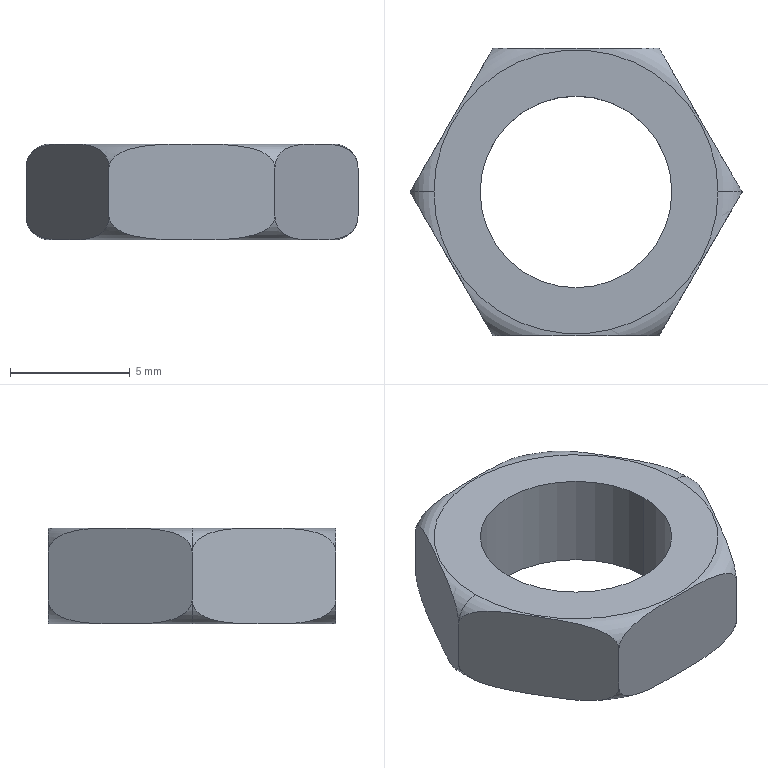Component | SolidWorks | F-YBXFJFA-RB0806-1_F-YBXFJFA-RB0806_Rb-Nut-2 | 1 solid | 14 faces | box 13.86 x 12 x 4 mm | volume 296 mm3 | plane 8 | torus 4 | cylinder 2 | commonest cylinder face diameters 8 x2
STEP:
#1=COLOUR_RGB('',0.7922,0.8196,0.9333);
#2=FILL_AREA_STYLE_COLOUR('',#1);
#3=FILL_AREA_STYLE('',(#2));
#4=SURFACE_STYLE_FILL_AREA(#3);
#5=SURFACE_SIDE_STYLE('',(#4));
#6=SURFACE_STYLE_USAGE(.BOTH.,#5);
#7=PRESENTATION_STYLE_ASSIGNMENT((#6));
#8=CARTESIAN_POINT('',(10.954,12.172,1.83));
#9=VERTEX_POINT('',#8);
#10=CARTESIAN_POINT('',(10.487,12.172,1.83));
#11=VERTEX_POINT('',#10);
#12=CARTESIAN_POINT('',(10.721,12.172,1.83));
#13=DIRECTION('',(0.,0.,1.));
#14=DIRECTION('',(1.,0.,0.));
#15=AXIS2_PLACEMENT_3D('',#12,#13,#14);
#16=CIRCLE('',#15,0.2334);
#17=EDGE_CURVE('',#9,#11,#16,.T.);
#18=ORIENTED_EDGE('',*,*,#17,.T.);
#19=CARTESIAN_POINT('',(10.448,12.172,1.869));
#20=VERTEX_POINT('',#19);
#21=CARTESIAN_POINT('',(10.487,12.172,1.869));
#22=DIRECTION('',(0.,1.,0.));
#23=DIRECTION('',(-1.,0.,0.));
#24=AXIS2_PLACEMENT_3D('',#21,#22,#23);
#25=CIRCLE('',#24,0.03937);
#26=EDGE_CURVE('',#11,#20,#25,.T.);
#27=ORIENTED_EDGE('',*,*,#26,.T.);
#28=CARTESIAN_POINT('',(10.584,12.408,1.869));
#29=VERTEX_POINT('',#28);
#30=CARTESIAN_POINT('',(10.448,12.172,1.869));
#31=CARTESIAN_POINT('',(10.448,12.172,1.866));
#32=CARTESIAN_POINT('',(10.448,12.173,1.863));
#33=CARTESIAN_POINT('',(10.45,12.175,1.857));
#34=CARTESIAN_POINT('',(10.451,12.177,1.854));
#35=CARTESIAN_POINT('',(10.453,12.181,1.85));
#36=CARTESIAN_POINT('',(10.454,12.183,1.848));
#37=CARTESIAN_POINT('',(10.457,12.188,1.845));
#38=CARTESIAN_POINT('',(10.458,12.19,1.843));
#39=CARTESIAN_POINT('',(10.463,12.198,1.839));
#40=CARTESIAN_POINT('',(10.466,12.203,1.837));
#41=CARTESIAN_POINT('',(10.472,12.214,1.835));
#42=CARTESIAN_POINT('',(10.475,12.219,1.833));
#43=CARTESIAN_POINT('',(10.484,12.236,1.831));
#44=CARTESIAN_POINT('',(10.491,12.247,1.831));
#45=CARTESIAN_POINT('',(10.503,12.269,1.83));
#46=CARTESIAN_POINT('',(10.51,12.28,1.83));
#47=CARTESIAN_POINT('',(10.523,12.301,1.83));
#48=CARTESIAN_POINT('',(10.529,12.312,1.83));
#49=CARTESIAN_POINT('',(10.542,12.334,1.831));
#50=CARTESIAN_POINT('',(10.548,12.345,1.831));
#51=CARTESIAN_POINT('',(10.557,12.362,1.834));
#52=CARTESIAN_POINT('',(10.56,12.367,1.835));
#53=CARTESIAN_POINT('',(10.567,12.378,1.837));
#54=CARTESIAN_POINT('',(10.57,12.383,1.839));
#55=CARTESIAN_POINT('',(10.575,12.393,1.845));
#56=CARTESIAN_POINT('',(10.578,12.398,1.848));
#57=CARTESIAN_POINT('',(10.582,12.404,1.855));
#58=CARTESIAN_POINT('',(10.582,12.405,1.857));
#59=CARTESIAN_POINT('',(10.584,12.408,1.863));
#60=CARTESIAN_POINT('',(10.584,12.408,1.866));
#61=CARTESIAN_POINT('',(10.584,12.408,1.869));
#62=B_SPLINE_CURVE_WITH_KNOTS('',3,(#30,#31,#32,#33,#34,#35,#36,#37,#38,#39,#40,#41,#42,#43,#44,#45,#46,#47,#48,#49,#50,#51,#52,#53,#54,#55,#56,#57,#58,#59,#60,#61),.UNSPECIFIED.,.F.,.F.,(4,2,2,2,2,2,2,2,2,2,2,2,2,2,2,4),(0.0000002,0.0002437,0.0004871,0.0007306,0.0009741,0.001461,0.001948,0.002922,0.003896,0.00487,0.005843,0.00633,0.006817,0.007304,0.007548,0.007791),.UNSPECIFIED.);
#63=EDGE_CURVE('',#20,#29,#62,.T.);
#64=ORIENTED_EDGE('',*,*,#63,.T.);
#65=CARTESIAN_POINT('',(10.857,12.408,1.869));
#66=VERTEX_POINT('',#65);
#67=CARTESIAN_POINT('',(10.584,12.408,1.869));
#68=CARTESIAN_POINT('',(10.584,12.408,1.866));
#69=CARTESIAN_POINT('',(10.585,12.408,1.863));
#70=CARTESIAN_POINT('',(10.588,12.408,1.857));
#71=CARTESIAN_POINT('',(10.59,12.408,1.855));
#72=CARTESIAN_POINT('',(10.594,12.408,1.85));
#73=CARTESIAN_POINT('',(10.597,12.408,1.848));
#74=CARTESIAN_POINT('',(10.602,12.408,1.845));
#75=CARTESIAN_POINT('',(10.605,12.408,1.843));
#76=CARTESIAN_POINT('',(10.614,12.408,1.839));
#77=CARTESIAN_POINT('',(10.62,12.408,1.837));
#78=CARTESIAN_POINT('',(10.632,12.408,1.835));
#79=CARTESIAN_POINT('',(10.638,12.408,1.834));
#80=CARTESIAN_POINT('',(10.657,12.408,1.831));
#81=CARTESIAN_POINT('',(10.67,12.408,1.831));
#82=CARTESIAN_POINT('',(10.695,12.408,1.83));
#83=CARTESIAN_POINT('',(10.708,12.408,1.83));
#84=CARTESIAN_POINT('',(10.733,12.408,1.83));
#85=CARTESIAN_POINT('',(10.746,12.408,1.83));
#86=CARTESIAN_POINT('',(10.771,12.408,1.831));
#87=CARTESIAN_POINT('',(10.784,12.408,1.831));
#88=CARTESIAN_POINT('',(10.803,12.408,1.833));
#89=CARTESIAN_POINT('',(10.809,12.408,1.835));
#90=CARTESIAN_POINT('',(10.821,12.408,1.837));
#91=CARTESIAN_POINT('',(10.827,12.408,1.839));
#92=CARTESIAN_POINT('',(10.839,12.408,1.844));
#93=CARTESIAN_POINT('',(10.845,12.408,1.848));
#94=CARTESIAN_POINT('',(10.851,12.408,1.854));
#95=CARTESIAN_POINT('',(10.853,12.408,1.857));
#96=CARTESIAN_POINT('',(10.856,12.408,1.863));
#97=CARTESIAN_POINT('',(10.857,12.408,1.866));
#98=CARTESIAN_POINT('',(10.857,12.408,1.869));
#99=B_SPLINE_CURVE_WITH_KNOTS('',3,(#67,#68,#69,#70,#71,#72,#73,#74,#75,#76,#77,#78,#79,#80,#81,#82,#83,#84,#85,#86,#87,#88,#89,#90,#91,#92,#93,#94,#95,#96,#97,#98),.UNSPECIFIED.,.F.,.F.,(4,2,2,2,2,2,2,2,2,2,2,2,2,2,2,4),(0.01157,0.01181,0.01205,0.01229,0.01253,0.01302,0.0135,0.01446,0.01543,0.0164,0.01736,0.01784,0.01833,0.01881,0.01905,0.01929),.UNSPECIFIED.);
#100=EDGE_CURVE('',#29,#66,#99,.T.);
#101=ORIENTED_EDGE('',*,*,#100,.T.);
#102=CARTESIAN_POINT('',(10.993,12.172,1.869));
#103=VERTEX_POINT('',#102);
#104=CARTESIAN_POINT('',(10.857,12.408,1.869));
#105=CARTESIAN_POINT('',(10.857,12.408,1.866));
#106=CARTESIAN_POINT('',(10.857,12.408,1.863));
#107=CARTESIAN_POINT('',(10.859,12.405,1.857));
#108=CARTESIAN_POINT('',(10.86,12.404,1.854));
#109=CARTESIAN_POINT('',(10.862,12.4,1.85));
#110=CARTESIAN_POINT('',(10.863,12.397,1.848));
#111=CARTESIAN_POINT('',(10.866,12.393,1.845));
#112=CARTESIAN_POINT('',(10.868,12.39,1.843));
#113=CARTESIAN_POINT('',(10.872,12.383,1.839));
#114=CARTESIAN_POINT('',(10.875,12.377,1.837));
#115=CARTESIAN_POINT('',(10.881,12.367,1.835));
#116=CARTESIAN_POINT('',(10.884,12.361,1.833));
#117=CARTESIAN_POINT('',(10.894,12.345,1.831));
#118=CARTESIAN_POINT('',(10.9,12.334,1.831));
#119=CARTESIAN_POINT('',(10.913,12.312,1.83));
#120=CARTESIAN_POINT('',(10.919,12.301,1.83));
#121=CARTESIAN_POINT('',(10.932,12.279,1.83));
#122=CARTESIAN_POINT('',(10.938,12.268,1.83));
#123=CARTESIAN_POINT('',(10.951,12.246,1.831));
#124=CARTESIAN_POINT('',(10.957,12.235,1.831));
#125=CARTESIAN_POINT('',(10.966,12.219,1.834));
#126=CARTESIAN_POINT('',(10.97,12.214,1.835));
#127=CARTESIAN_POINT('',(10.976,12.203,1.837));
#128=CARTESIAN_POINT('',(10.979,12.198,1.839));
#129=CARTESIAN_POINT('',(10.985,12.188,1.845));
#130=CARTESIAN_POINT('',(10.987,12.183,1.848));
#131=CARTESIAN_POINT('',(10.991,12.177,1.855));
#132=CARTESIAN_POINT('',(10.992,12.175,1.857));
#133=CARTESIAN_POINT('',(10.993,12.173,1.863));
#134=CARTESIAN_POINT('',(10.993,12.172,1.866));
#135=CARTESIAN_POINT('',(10.993,12.172,1.869));
#136=B_SPLINE_CURVE_WITH_KNOTS('',3,(#104,#105,#106,#107,#108,#109,#110,#111,#112,#113,#114,#115,#116,#117,#118,#119,#120,#121,#122,#123,#124,#125,#126,#127,#128,#129,#130,#131,#132,#133,#134,#135),.UNSPECIFIED.,.F.,.F.,(4,2,2,2,2,2,2,2,2,2,2,2,2,2,2,4),(0.0000002,0.0002437,0.0004871,0.0007306,0.0009741,0.001461,0.001948,0.002922,0.003896,0.00487,0.005843,0.00633,0.006817,0.007304,0.007548,0.007791),.UNSPECIFIED.);
#137=EDGE_CURVE('',#66,#103,#136,.T.);
#138=ORIENTED_EDGE('',*,*,#137,.T.);
#139=CARTESIAN_POINT('',(10.954,12.172,1.869));
#140=DIRECTION('',(0.,-1.,0.));
#141=DIRECTION('',(0.,0.,-1.));
#142=AXIS2_PLACEMENT_3D('',#139,#140,#141);
#143=CIRCLE('',#142,0.03937);
#144=EDGE_CURVE('',#9,#103,#143,.T.);
#145=ORIENTED_EDGE('',*,*,#144,.F.);
#146=EDGE_LOOP('',(#18,#27,#64,#101,#138,#145));
#147=FACE_OUTER_BOUND('',#146,.T.);
#148=CARTESIAN_POINT('',(10.721,12.172,1.869));
#149=DIRECTION('',(0.,0.,1.));
#150=DIRECTION('',(1.,0.,0.));
#151=AXIS2_PLACEMENT_3D('',#148,#149,#150);
#152=TOROIDAL_SURFACE('',#151,0.2334,0.03937);
#153=ADVANCED_FACE('',(#147),#152,.T.);
#154=CARTESIAN_POINT('',(10.584,12.408,1.948));
#155=VERTEX_POINT('',#154);
#156=CARTESIAN_POINT('',(10.448,12.172,1.948));
#157=VERTEX_POINT('',#156);
#158=CARTESIAN_POINT('',(10.584,12.408,1.948));
#159=CARTESIAN_POINT('',(10.584,12.408,1.951));
#160=CARTESIAN_POINT('',(10.584,12.408,1.954));
#161=CARTESIAN_POINT('',(10.582,12.405,1.96));
#162=CARTESIAN_POINT('',(10.581,12.404,1.963));
#163=CARTESIAN_POINT('',(10.579,12.4,1.967));
#164=CARTESIAN_POINT('',(10.578,12.397,1.969));
#165=CARTESIAN_POINT('',(10.575,12.393,1.973));
#166=CARTESIAN_POINT('',(10.574,12.39,1.974));
#167=CARTESIAN_POINT('',(10.569,12.383,1.978));
#168=CARTESIAN_POINT('',(10.566,12.377,1.98));
#169=CARTESIAN_POINT('',(10.56,12.367,1.983));
#170=CARTESIAN_POINT('',(10.557,12.361,1.984));
#171=CARTESIAN_POINT('',(10.548,12.345,1.986));
#172=CARTESIAN_POINT('',(10.541,12.334,1.987));
#173=CARTESIAN_POINT('',(10.529,12.312,1.987));
#174=CARTESIAN_POINT('',(10.522,12.301,1.987));
#175=CARTESIAN_POINT('',(10.51,12.279,1.987));
#176=CARTESIAN_POINT('',(10.503,12.268,1.987));
#177=CARTESIAN_POINT('',(10.491,12.246,1.987));
#178=CARTESIAN_POINT('',(10.484,12.235,1.986));
#179=CARTESIAN_POINT('',(10.475,12.219,1.984));
#180=CARTESIAN_POINT('',(10.472,12.214,1.983));
#181=CARTESIAN_POINT('',(10.466,12.203,1.98));
#182=CARTESIAN_POINT('',(10.463,12.198,1.978));
#183=CARTESIAN_POINT('',(10.457,12.188,1.973));
#184=CARTESIAN_POINT('',(10.454,12.183,1.969));
#185=CARTESIAN_POINT('',(10.451,12.177,1.963));
#186=CARTESIAN_POINT('',(10.45,12.175,1.96));
#187=CARTESIAN_POINT('',(10.448,12.173,1.954));
#188=CARTESIAN_POINT('',(10.448,12.172,1.951));
#189=CARTESIAN_POINT('',(10.448,12.172,1.948));
#190=B_SPLINE_CURVE_WITH_KNOTS('',3,(#158,#159,#160,#161,#162,#163,#164,#165,#166,#167,#168,#169,#170,#171,#172,#173,#174,#175,#176,#177,#178,#179,#180,#181,#182,#183,#184,#185,#186,#187,#188,#189),.UNSPECIFIED.,.F.,.F.,(4,2,2,2,2,2,2,2,2,2,2,2,2,2,2,4),(0.0000002,0.0002437,0.0004871,0.0007306,0.0009741,0.001461,0.001948,0.002922,0.003896,0.00487,0.005843,0.00633,0.006817,0.007304,0.007548,0.007791),.UNSPECIFIED.);
#191=EDGE_CURVE('',#155,#157,#190,.T.);
#192=ORIENTED_EDGE('',*,*,#191,.T.);
#193=CARTESIAN_POINT('',(10.487,12.172,1.987));
#194=VERTEX_POINT('',#193);
#195=CARTESIAN_POINT('',(10.487,12.172,1.948));
#196=DIRECTION('',(0.,1.,0.));
#197=DIRECTION('',(-1.,0.,0.));
#198=AXIS2_PLACEMENT_3D('',#195,#196,#197);
#199=CIRCLE('',#198,0.03937);
#200=EDGE_CURVE('',#157,#194,#199,.T.);
#201=ORIENTED_EDGE('',*,*,#200,.T.);
#202=CARTESIAN_POINT('',(10.954,12.172,1.987));
#203=VERTEX_POINT('',#202);
#204=CARTESIAN_POINT('',(10.721,12.172,1.987));
#205=DIRECTION('',(0.,0.,1.));
#206=DIRECTION('',(1.,0.,0.));
#207=AXIS2_PLACEMENT_3D('',#204,#205,#206);
#208=CIRCLE('',#207,0.2334);
#209=EDGE_CURVE('',#203,#194,#208,.T.);
#210=ORIENTED_EDGE('',*,*,#209,.F.);
#211=CARTESIAN_POINT('',(10.993,12.172,1.948));
#212=VERTEX_POINT('',#211);
#213=CARTESIAN_POINT('',(10.954,12.172,1.948));
#214=DIRECTION('',(0.,-1.,0.));
#215=DIRECTION('',(0.,0.,-1.));
#216=AXIS2_PLACEMENT_3D('',#213,#214,#215);
#217=CIRCLE('',#216,0.03937);
#218=EDGE_CURVE('',#212,#203,#217,.T.);
#219=ORIENTED_EDGE('',*,*,#218,.F.);
#220=CARTESIAN_POINT('',(10.857,12.408,1.948));
#221=VERTEX_POINT('',#220);
#222=CARTESIAN_POINT('',(10.993,12.172,1.948));
#223=CARTESIAN_POINT('',(10.993,12.172,1.951));
#224=CARTESIAN_POINT('',(10.993,12.173,1.954));
#225=CARTESIAN_POINT('',(10.992,12.175,1.96));
#226=CARTESIAN_POINT('',(10.991,12.177,1.963));
#227=CARTESIAN_POINT('',(10.988,12.181,1.967));
#228=CARTESIAN_POINT('',(10.987,12.183,1.969));
#229=CARTESIAN_POINT('',(10.984,12.188,1.973));
#230=CARTESIAN_POINT('',(10.983,12.19,1.974));
#231=CARTESIAN_POINT('',(10.979,12.198,1.978));
#232=CARTESIAN_POINT('',(10.976,12.203,1.98));
#233=CARTESIAN_POINT('',(10.969,12.214,1.983));
#234=CARTESIAN_POINT('',(10.966,12.219,1.984));
#235=CARTESIAN_POINT('',(10.957,12.236,1.986));
#236=CARTESIAN_POINT('',(10.951,12.247,1.987));
#237=CARTESIAN_POINT('',(10.938,12.269,1.987));
#238=CARTESIAN_POINT('',(10.932,12.28,1.987));
#239=CARTESIAN_POINT('',(10.919,12.301,1.987));
#240=CARTESIAN_POINT('',(10.913,12.312,1.987));
#241=CARTESIAN_POINT('',(10.9,12.334,1.987));
#242=CARTESIAN_POINT('',(10.894,12.345,1.986));
#243=CARTESIAN_POINT('',(10.884,12.362,1.984));
#244=CARTESIAN_POINT('',(10.881,12.367,1.983));
#245=CARTESIAN_POINT('',(10.875,12.378,1.98));
#246=CARTESIAN_POINT('',(10.872,12.383,1.978));
#247=CARTESIAN_POINT('',(10.866,12.393,1.973));
#248=CARTESIAN_POINT('',(10.863,12.398,1.969));
#249=CARTESIAN_POINT('',(10.86,12.404,1.963));
#250=CARTESIAN_POINT('',(10.859,12.405,1.96));
#251=CARTESIAN_POINT('',(10.857,12.408,1.954));
#252=CARTESIAN_POINT('',(10.857,12.408,1.951));
#253=CARTESIAN_POINT('',(10.857,12.408,1.948));
#254=B_SPLINE_CURVE_WITH_KNOTS('',3,(#222,#223,#224,#225,#226,#227,#228,#229,#230,#231,#232,#233,#234,#235,#236,#237,#238,#239,#240,#241,#242,#243,#244,#245,#246,#247,#248,#249,#250,#251,#252,#253),.UNSPECIFIED.,.F.,.F.,(4,2,2,2,2,2,2,2,2,2,2,2,2,2,2,4),(0.0000002,0.0002437,0.0004871,0.0007306,0.0009741,0.001461,0.001948,0.002922,0.003896,0.00487,0.005843,0.00633,0.006817,0.007304,0.007548,0.007791),.UNSPECIFIED.);
#255=EDGE_CURVE('',#212,#221,#254,.T.);
#256=ORIENTED_EDGE('',*,*,#255,.T.);
#257=CARTESIAN_POINT('',(10.857,12.408,1.948));
#258=CARTESIAN_POINT('',(10.857,12.408,1.951));
#259=CARTESIAN_POINT('',(10.856,12.408,1.954));
#260=CARTESIAN_POINT('',(10.853,12.408,1.96));
#261=CARTESIAN_POINT('',(10.851,12.408,1.963));
#262=CARTESIAN_POINT('',(10.847,12.408,1.967));
#263=CARTESIAN_POINT('',(10.844,12.408,1.969));
#264=CARTESIAN_POINT('',(10.839,12.408,1.973));
#265=CARTESIAN_POINT('',(10.836,12.408,1.974));
#266=CARTESIAN_POINT('',(10.828,12.408,1.978));
#267=CARTESIAN_POINT('',(10.821,12.408,1.98));
#268=CARTESIAN_POINT('',(10.809,12.408,1.983));
#269=CARTESIAN_POINT('',(10.803,12.408,1.984));
#270=CARTESIAN_POINT('',(10.784,12.408,1.986));
#271=CARTESIAN_POINT('',(10.772,12.408,1.987));
#272=CARTESIAN_POINT('',(10.746,12.408,1.987));
#273=CARTESIAN_POINT('',(10.734,12.408,1.987));
#274=CARTESIAN_POINT('',(10.708,12.408,1.987));
#275=CARTESIAN_POINT('',(10.696,12.408,1.987));
#276=CARTESIAN_POINT('',(10.67,12.408,1.987));
#277=CARTESIAN_POINT('',(10.658,12.408,1.986));
#278=CARTESIAN_POINT('',(10.639,12.408,1.984));
#279=CARTESIAN_POINT('',(10.632,12.408,1.983));
#280=CARTESIAN_POINT('',(10.62,12.408,1.98));
#281=CARTESIAN_POINT('',(10.614,12.408,1.978));
#282=CARTESIAN_POINT('',(10.602,12.408,1.973));
#283=CARTESIAN_POINT('',(10.597,12.408,1.97));
#284=CARTESIAN_POINT('',(10.59,12.408,1.963));
#285=CARTESIAN_POINT('',(10.588,12.408,1.96));
#286=CARTESIAN_POINT('',(10.585,12.408,1.954));
#287=CARTESIAN_POINT('',(10.584,12.408,1.951));
#288=CARTESIAN_POINT('',(10.584,12.408,1.948));
#289=B_SPLINE_CURVE_WITH_KNOTS('',3,(#257,#258,#259,#260,#261,#262,#263,#264,#265,#266,#267,#268,#269,#270,#271,#272,#273,#274,#275,#276,#277,#278,#279,#280,#281,#282,#283,#284,#285,#286,#287,#288),.UNSPECIFIED.,.F.,.F.,(4,2,2,2,2,2,2,2,2,2,2,2,2,2,2,4),(0.01157,0.01181,0.01205,0.01229,0.01253,0.01302,0.0135,0.01446,0.01543,0.0164,0.01736,0.01784,0.01833,0.01881,0.01905,0.01929),.UNSPECIFIED.);
#290=EDGE_CURVE('',#221,#155,#289,.T.);
#291=ORIENTED_EDGE('',*,*,#290,.T.);
#292=EDGE_LOOP('',(#192,#201,#210,#219,#256,#291));
#293=FACE_OUTER_BOUND('',#292,.T.);
#294=CARTESIAN_POINT('',(10.721,12.172,1.948));
#295=DIRECTION('',(0.,0.,1.));
#296=DIRECTION('',(1.,0.,0.));
#297=AXIS2_PLACEMENT_3D('',#294,#295,#296);
#298=TOROIDAL_SURFACE('',#297,0.2334,0.03937);
#299=ADVANCED_FACE('',(#293),#298,.T.);
#300=CARTESIAN_POINT('',(10.563,12.172,1.987));
#301=VERTEX_POINT('',#300);
#302=CARTESIAN_POINT('',(10.878,12.172,1.987));
#303=VERTEX_POINT('',#302);
#304=CARTESIAN_POINT('',(10.721,12.172,1.987));
#305=DIRECTION('',(0.,0.,1.));
#306=DIRECTION('',(1.,0.,0.));
#307=AXIS2_PLACEMENT_3D('',#304,#305,#306);
#308=CIRCLE('',#307,0.1575);
#309=EDGE_CURVE('',#301,#303,#308,.T.);
#310=ORIENTED_EDGE('',*,*,#309,.T.);
#311=CARTESIAN_POINT('',(10.878,12.172,1.83));
#312=VERTEX_POINT('',#311);
#313=CARTESIAN_POINT('',(10.878,12.172,1.987));
#314=DIRECTION('',(0.,0.,-1.));
#315=VECTOR('',#314,39.37);
#316=LINE('',#313,#315);
#317=EDGE_CURVE('',#303,#312,#316,.T.);
#318=ORIENTED_EDGE('',*,*,#317,.T.);
#319=CARTESIAN_POINT('',(10.563,12.172,1.83));
#320=VERTEX_POINT('',#319);
#321=CARTESIAN_POINT('',(10.721,12.172,1.83));
#322=DIRECTION('',(0.,0.,1.));
#323=DIRECTION('',(1.,0.,0.));
#324=AXIS2_PLACEMENT_3D('',#321,#322,#323);
#325=CIRCLE('',#324,0.1575);
#326=EDGE_CURVE('',#320,#312,#325,.T.);
#327=ORIENTED_EDGE('',*,*,#326,.F.);
#328=CARTESIAN_POINT('',(10.563,12.172,1.987));
#329=DIRECTION('',(0.,0.,-1.));
#330=VECTOR('',#329,39.37);
#331=LINE('',#328,#330);
#332=EDGE_CURVE('',#301,#320,#331,.T.);
#333=ORIENTED_EDGE('',*,*,#332,.F.);
#334=EDGE_LOOP('',(#310,#318,#327,#333));
#335=FACE_OUTER_BOUND('',#334,.T.);
#336=CARTESIAN_POINT('',(10.721,12.172,1.987));
#337=DIRECTION('',(0.,0.,-1.));
#338=DIRECTION('',(-1.,0.,0.));
#339=AXIS2_PLACEMENT_3D('',#336,#337,#338);
#340=CYLINDRICAL_SURFACE('',#339,0.1575);
#341=ADVANCED_FACE('',(#335),#340,.F.);
#342=CARTESIAN_POINT('',(10.857,11.936,1.869));
#343=VERTEX_POINT('',#342);
#344=CARTESIAN_POINT('',(10.993,12.172,1.869));
#345=CARTESIAN_POINT('',(10.993,12.172,1.866));
#346=CARTESIAN_POINT('',(10.993,12.172,1.863));
#347=CARTESIAN_POINT('',(10.992,12.169,1.857));
#348=CARTESIAN_POINT('',(10.991,12.167,1.854));
#349=CARTESIAN_POINT('',(10.988,12.163,1.85));
#350=CARTESIAN_POINT('',(10.987,12.161,1.848));
#351=CARTESIAN_POINT('',(10.984,12.157,1.845));
#352=CARTESIAN_POINT('',(10.983,12.154,1.843));
#353=CARTESIAN_POINT('',(10.979,12.147,1.839));
#354=CARTESIAN_POINT('',(10.976,12.141,1.837));
#355=CARTESIAN_POINT('',(10.969,12.131,1.835));
#356=CARTESIAN_POINT('',(10.966,12.125,1.833));
#357=CARTESIAN_POINT('',(10.957,12.109,1.831));
#358=CARTESIAN_POINT('',(10.951,12.098,1.831));
#359=CARTESIAN_POINT('',(10.938,12.076,1.83));
#360=CARTESIAN_POINT('',(10.932,12.065,1.83));
#361=CARTESIAN_POINT('',(10.919,12.043,1.83));
#362=CARTESIAN_POINT('',(10.913,12.032,1.83));
#363=CARTESIAN_POINT('',(10.9,12.01,1.831));
#364=CARTESIAN_POINT('',(10.894,11.999,1.831));
#365=CARTESIAN_POINT('',(10.884,11.983,1.834));
#366=CARTESIAN_POINT('',(10.881,11.977,1.835));
#367=CARTESIAN_POINT('',(10.875,11.967,1.837));
#368=CARTESIAN_POINT('',(10.872,11.962,1.839));
#369=CARTESIAN_POINT('',(10.866,11.951,1.845));
#370=CARTESIAN_POINT('',(10.863,11.947,1.848));
#371=CARTESIAN_POINT('',(10.86,11.941,1.855));
#372=CARTESIAN_POINT('',(10.859,11.939,1.857));
#373=CARTESIAN_POINT('',(10.857,11.937,1.863));
#374=CARTESIAN_POINT('',(10.857,11.936,1.866));
#375=CARTESIAN_POINT('',(10.857,11.936,1.869));
#376=B_SPLINE_CURVE_WITH_KNOTS('',3,(#344,#345,#346,#347,#348,#349,#350,#351,#352,#353,#354,#355,#356,#357,#358,#359,#360,#361,#362,#363,#364,#365,#366,#367,#368,#369,#370,#371,#372,#373,#374,#375),.UNSPECIFIED.,.F.,.F.,(4,2,2,2,2,2,2,2,2,2,2,2,2,2,2,4),(0.0000002,0.0002437,0.0004871,0.0007306,0.0009741,0.001461,0.001948,0.002922,0.003896,0.00487,0.005843,0.00633,0.006817,0.007304,0.007548,0.007791),.UNSPECIFIED.);
#377=EDGE_CURVE('',#103,#343,#376,.T.);
#378=ORIENTED_EDGE('',*,*,#377,.F.);
#379=CARTESIAN_POINT('',(10.993,12.172,1.987));
#380=DIRECTION('',(0.,0.,-1.));
#381=VECTOR('',#380,39.37);
#382=LINE('',#379,#381);
#383=EDGE_CURVE('',#212,#103,#382,.T.);
#384=ORIENTED_EDGE('',*,*,#383,.F.);
#385=CARTESIAN_POINT('',(10.857,11.936,1.948));
#386=VERTEX_POINT('',#385);
#387=CARTESIAN_POINT('',(10.857,11.936,1.948));
#388=CARTESIAN_POINT('',(10.857,11.936,1.951));
#389=CARTESIAN_POINT('',(10.857,11.937,1.954));
#390=CARTESIAN_POINT('',(10.859,11.939,1.96));
#391=CARTESIAN_POINT('',(10.86,11.941,1.963));
#392=CARTESIAN_POINT('',(10.862,11.945,1.967));
#393=CARTESIAN_POINT('',(10.863,11.947,1.969));
#394=CARTESIAN_POINT('',(10.866,11.952,1.973));
#395=CARTESIAN_POINT('',(10.868,11.954,1.974));
#396=CARTESIAN_POINT('',(10.872,11.962,1.978));
#397=CARTESIAN_POINT('',(10.875,11.967,1.98));
#398=CARTESIAN_POINT('',(10.881,11.978,1.983));
#399=CARTESIAN_POINT('',(10.884,11.983,1.984));
#400=CARTESIAN_POINT('',(10.894,11.999,1.986));
#401=CARTESIAN_POINT('',(10.9,12.01,1.987));
#402=CARTESIAN_POINT('',(10.913,12.032,1.987));
#403=CARTESIAN_POINT('',(10.919,12.043,1.987));
#404=CARTESIAN_POINT('',(10.932,12.065,1.987));
#405=CARTESIAN_POINT('',(10.938,12.076,1.987));
#406=CARTESIAN_POINT('',(10.951,12.098,1.987));
#407=CARTESIAN_POINT('',(10.957,12.109,1.986));
#408=CARTESIAN_POINT('',(10.966,12.125,1.984));
#409=CARTESIAN_POINT('',(10.97,12.131,1.983));
#410=CARTESIAN_POINT('',(10.976,12.142,1.98));
#411=CARTESIAN_POINT('',(10.979,12.147,1.978));
#412=CARTESIAN_POINT('',(10.985,12.157,1.973));
#413=CARTESIAN_POINT('',(10.987,12.162,1.969));
#414=CARTESIAN_POINT('',(10.991,12.167,1.963));
#415=CARTESIAN_POINT('',(10.992,12.169,1.96));
#416=CARTESIAN_POINT('',(10.993,12.172,1.954));
#417=CARTESIAN_POINT('',(10.993,12.172,1.951));
#418=CARTESIAN_POINT('',(10.993,12.172,1.948));
#419=B_SPLINE_CURVE_WITH_KNOTS('',3,(#387,#388,#389,#390,#391,#392,#393,#394,#395,#396,#397,#398,#399,#400,#401,#402,#403,#404,#405,#406,#407,#408,#409,#410,#411,#412,#413,#414,#415,#416,#417,#418),.UNSPECIFIED.,.F.,.F.,(4,2,2,2,2,2,2,2,2,2,2,2,2,2,2,4),(0.0000002,0.0002437,0.0004871,0.0007306,0.0009741,0.001461,0.001948,0.002922,0.003896,0.00487,0.005843,0.00633,0.006817,0.007304,0.007548,0.007791),.UNSPECIFIED.);
#420=EDGE_CURVE('',#386,#212,#419,.T.);
#421=ORIENTED_EDGE('',*,*,#420,.F.);
#422=CARTESIAN_POINT('',(10.857,11.936,1.987));
#423=DIRECTION('',(0.,0.,-1.));
#424=VECTOR('',#423,39.37);
#425=LINE('',#422,#424);
#426=EDGE_CURVE('',#386,#343,#425,.T.);
#427=ORIENTED_EDGE('',*,*,#426,.T.);
#428=EDGE_LOOP('',(#378,#384,#421,#427));
#429=FACE_OUTER_BOUND('',#428,.T.);
#430=CARTESIAN_POINT('',(10.857,11.936,1.987));
#431=DIRECTION('',(-0.866,0.5,0.));
#432=DIRECTION('',(-0.5,-0.866,0.));
#433=AXIS2_PLACEMENT_3D('',#430,#431,#432);
#434=PLANE('',#433);
#435=ADVANCED_FACE('',(#429),#434,.F.);
#436=ORIENTED_EDGE('',*,*,#137,.F.);
#437=CARTESIAN_POINT('',(10.857,12.408,1.987));
#438=DIRECTION('',(0.,0.,-1.));
#439=VECTOR('',#438,39.37);
#440=LINE('',#437,#439);
#441=EDGE_CURVE('',#221,#66,#440,.T.);
#442=ORIENTED_EDGE('',*,*,#441,.F.);
#443=ORIENTED_EDGE('',*,*,#255,.F.);
#444=ORIENTED_EDGE('',*,*,#383,.T.);
#445=EDGE_LOOP('',(#436,#442,#443,#444));
#446=FACE_OUTER_BOUND('',#445,.T.);
#447=CARTESIAN_POINT('',(10.993,12.172,1.987));
#448=DIRECTION('',(-0.866,-0.5,0.));
#449=DIRECTION('',(0.5,-0.866,0.));
#450=AXIS2_PLACEMENT_3D('',#447,#448,#449);
#451=PLANE('',#450);
#452=ADVANCED_FACE('',(#446),#451,.F.);
#453=ORIENTED_EDGE('',*,*,#100,.F.);
#454=CARTESIAN_POINT('',(10.584,12.408,1.987));
#455=DIRECTION('',(0.,0.,-1.));
#456=VECTOR('',#455,39.37);
#457=LINE('',#454,#456);
#458=EDGE_CURVE('',#155,#29,#457,.T.);
#459=ORIENTED_EDGE('',*,*,#458,.F.);
#460=ORIENTED_EDGE('',*,*,#290,.F.);
#461=ORIENTED_EDGE('',*,*,#441,.T.);
#462=EDGE_LOOP('',(#453,#459,#460,#461));
#463=FACE_OUTER_BOUND('',#462,.T.);
#464=CARTESIAN_POINT('',(10.857,12.408,1.987));
#465=DIRECTION('',(0.,-1.,0.));
#466=DIRECTION('',(0.,0.,-1.));
#467=AXIS2_PLACEMENT_3D('',#464,#465,#466);
#468=PLANE('',#467);
#469=ADVANCED_FACE('',(#463),#468,.F.);
#470=ORIENTED_EDGE('',*,*,#63,.F.);
#471=CARTESIAN_POINT('',(10.448,12.172,1.987));
#472=DIRECTION('',(0.,0.,-1.));
#473=VECTOR('',#472,39.37);
#474=LINE('',#471,#473);
#475=EDGE_CURVE('',#157,#20,#474,.T.);
#476=ORIENTED_EDGE('',*,*,#475,.F.);
#477=ORIENTED_EDGE('',*,*,#191,.F.);
#478=ORIENTED_EDGE('',*,*,#458,.T.);
#479=EDGE_LOOP('',(#470,#476,#477,#478));
#480=FACE_OUTER_BOUND('',#479,.T.);
#481=CARTESIAN_POINT('',(10.584,12.408,1.987));
#482=DIRECTION('',(0.866,-0.5,0.));
#483=DIRECTION('',(0.5,0.866,0.));
#484=AXIS2_PLACEMENT_3D('',#481,#482,#483);
#485=PLANE('',#484);
#486=ADVANCED_FACE('',(#480),#485,.F.);
#487=CARTESIAN_POINT('',(10.584,11.936,1.869));
#488=VERTEX_POINT('',#487);
#489=CARTESIAN_POINT('',(10.584,11.936,1.869));
#490=CARTESIAN_POINT('',(10.584,11.936,1.866));
#491=CARTESIAN_POINT('',(10.584,11.937,1.863));
#492=CARTESIAN_POINT('',(10.582,11.939,1.857));
#493=CARTESIAN_POINT('',(10.581,11.941,1.854));
#494=CARTESIAN_POINT('',(10.579,11.945,1.85));
#495=CARTESIAN_POINT('',(10.578,11.947,1.848));
#496=CARTESIAN_POINT('',(10.575,11.952,1.845));
#497=CARTESIAN_POINT('',(10.574,11.954,1.843));
#498=CARTESIAN_POINT('',(10.569,11.962,1.839));
#499=CARTESIAN_POINT('',(10.566,11.967,1.837));
#500=CARTESIAN_POINT('',(10.56,11.978,1.835));
#501=CARTESIAN_POINT('',(10.557,11.983,1.833));
#502=CARTESIAN_POINT('',(10.548,11.999,1.831));
#503=CARTESIAN_POINT('',(10.541,12.01,1.831));
#504=CARTESIAN_POINT('',(10.529,12.032,1.83));
#505=CARTESIAN_POINT('',(10.522,12.043,1.83));
#506=CARTESIAN_POINT('',(10.51,12.065,1.83));
#507=CARTESIAN_POINT('',(10.503,12.076,1.83));
#508=CARTESIAN_POINT('',(10.491,12.098,1.831));
#509=CARTESIAN_POINT('',(10.484,12.109,1.831));
#510=CARTESIAN_POINT('',(10.475,12.125,1.834));
#511=CARTESIAN_POINT('',(10.472,12.131,1.835));
#512=CARTESIAN_POINT('',(10.466,12.142,1.837));
#513=CARTESIAN_POINT('',(10.463,12.147,1.839));
#514=CARTESIAN_POINT('',(10.457,12.157,1.845));
#515=CARTESIAN_POINT('',(10.454,12.162,1.848));
#516=CARTESIAN_POINT('',(10.451,12.167,1.855));
#517=CARTESIAN_POINT('',(10.45,12.169,1.857));
#518=CARTESIAN_POINT('',(10.448,12.172,1.863));
#519=CARTESIAN_POINT('',(10.448,12.172,1.866));
#520=CARTESIAN_POINT('',(10.448,12.172,1.869));
#521=B_SPLINE_CURVE_WITH_KNOTS('',3,(#489,#490,#491,#492,#493,#494,#495,#496,#497,#498,#499,#500,#501,#502,#503,#504,#505,#506,#507,#508,#509,#510,#511,#512,#513,#514,#515,#516,#517,#518,#519,#520),.UNSPECIFIED.,.F.,.F.,(4,2,2,2,2,2,2,2,2,2,2,2,2,2,2,4),(0.0000002,0.0002437,0.0004871,0.0007306,0.0009741,0.001461,0.001948,0.002922,0.003896,0.00487,0.005843,0.00633,0.006817,0.007304,0.007548,0.007791),.UNSPECIFIED.);
#522=EDGE_CURVE('',#488,#20,#521,.T.);
#523=ORIENTED_EDGE('',*,*,#522,.F.);
#524=CARTESIAN_POINT('',(10.584,11.936,1.948));
#525=VERTEX_POINT('',#524);
#526=CARTESIAN_POINT('',(10.584,11.936,1.987));
#527=DIRECTION('',(0.,0.,-1.));
#528=VECTOR('',#527,39.37);
#529=LINE('',#526,#528);
#530=EDGE_CURVE('',#525,#488,#529,.T.);
#531=ORIENTED_EDGE('',*,*,#530,.F.);
#532=CARTESIAN_POINT('',(10.448,12.172,1.948));
#533=CARTESIAN_POINT('',(10.448,12.172,1.951));
#534=CARTESIAN_POINT('',(10.448,12.172,1.954));
#535=CARTESIAN_POINT('',(10.45,12.169,1.96));
#536=CARTESIAN_POINT('',(10.451,12.167,1.963));
#537=CARTESIAN_POINT('',(10.453,12.163,1.967));
#538=CARTESIAN_POINT('',(10.454,12.161,1.969));
#539=CARTESIAN_POINT('',(10.457,12.157,1.973));
#540=CARTESIAN_POINT('',(10.458,12.154,1.974));
#541=CARTESIAN_POINT('',(10.463,12.147,1.978));
#542=CARTESIAN_POINT('',(10.466,12.141,1.98));
#543=CARTESIAN_POINT('',(10.472,12.131,1.983));
#544=CARTESIAN_POINT('',(10.475,12.125,1.984));
#545=CARTESIAN_POINT('',(10.484,12.109,1.986));
#546=CARTESIAN_POINT('',(10.491,12.098,1.987));
#547=CARTESIAN_POINT('',(10.503,12.076,1.987));
#548=CARTESIAN_POINT('',(10.51,12.065,1.987));
#549=CARTESIAN_POINT('',(10.523,12.043,1.987));
#550=CARTESIAN_POINT('',(10.529,12.032,1.987));
#551=CARTESIAN_POINT('',(10.542,12.01,1.987));
#552=CARTESIAN_POINT('',(10.548,11.999,1.986));
#553=CARTESIAN_POINT('',(10.557,11.983,1.984));
#554=CARTESIAN_POINT('',(10.56,11.977,1.983));
#555=CARTESIAN_POINT('',(10.567,11.967,1.98));
#556=CARTESIAN_POINT('',(10.57,11.962,1.978));
#557=CARTESIAN_POINT('',(10.575,11.951,1.973));
#558=CARTESIAN_POINT('',(10.578,11.947,1.969));
#559=CARTESIAN_POINT('',(10.582,11.941,1.963));
#560=CARTESIAN_POINT('',(10.582,11.939,1.96));
#561=CARTESIAN_POINT('',(10.584,11.937,1.954));
#562=CARTESIAN_POINT('',(10.584,11.936,1.951));
#563=CARTESIAN_POINT('',(10.584,11.936,1.948));
#564=B_SPLINE_CURVE_WITH_KNOTS('',3,(#532,#533,#534,#535,#536,#537,#538,#539,#540,#541,#542,#543,#544,#545,#546,#547,#548,#549,#550,#551,#552,#553,#554,#555,#556,#557,#558,#559,#560,#561,#562,#563),.UNSPECIFIED.,.F.,.F.,(4,2,2,2,2,2,2,2,2,2,2,2,2,2,2,4),(0.0000002,0.0002437,0.0004871,0.0007306,0.0009741,0.001461,0.001948,0.002922,0.003896,0.00487,0.005843,0.00633,0.006817,0.007304,0.007548,0.007791),.UNSPECIFIED.);
#565=EDGE_CURVE('',#157,#525,#564,.T.);
#566=ORIENTED_EDGE('',*,*,#565,.F.);
#567=ORIENTED_EDGE('',*,*,#475,.T.);
#568=EDGE_LOOP('',(#523,#531,#566,#567));
#569=FACE_OUTER_BOUND('',#568,.T.);
#570=CARTESIAN_POINT('',(10.448,12.172,1.987));
#571=DIRECTION('',(0.866,0.5,0.));
#572=DIRECTION('',(-0.5,0.866,0.));
#573=AXIS2_PLACEMENT_3D('',#570,#571,#572);
#574=PLANE('',#573);
#575=ADVANCED_FACE('',(#569),#574,.F.);
#576=CARTESIAN_POINT('',(10.857,11.936,1.869));
#577=CARTESIAN_POINT('',(10.857,11.936,1.866));
#578=CARTESIAN_POINT('',(10.856,11.936,1.863));
#579=CARTESIAN_POINT('',(10.853,11.936,1.857));
#580=CARTESIAN_POINT('',(10.851,11.936,1.855));
#581=CARTESIAN_POINT('',(10.847,11.936,1.85));
#582=CARTESIAN_POINT('',(10.844,11.936,1.848));
#583=CARTESIAN_POINT('',(10.839,11.936,1.845));
#584=CARTESIAN_POINT('',(10.836,11.936,1.843));
#585=CARTESIAN_POINT('',(10.828,11.936,1.839));
#586=CARTESIAN_POINT('',(10.821,11.936,1.837));
#587=CARTESIAN_POINT('',(10.809,11.936,1.835));
#588=CARTESIAN_POINT('',(10.803,11.936,1.834));
#589=CARTESIAN_POINT('',(10.784,11.936,1.831));
#590=CARTESIAN_POINT('',(10.772,11.936,1.831));
#591=CARTESIAN_POINT('',(10.746,11.936,1.83));
#592=CARTESIAN_POINT('',(10.734,11.936,1.83));
#593=CARTESIAN_POINT('',(10.708,11.936,1.83));
#594=CARTESIAN_POINT('',(10.696,11.936,1.83));
#595=CARTESIAN_POINT('',(10.67,11.936,1.831));
#596=CARTESIAN_POINT('',(10.658,11.936,1.831));
#597=CARTESIAN_POINT('',(10.639,11.936,1.833));
#598=CARTESIAN_POINT('',(10.632,11.936,1.835));
#599=CARTESIAN_POINT('',(10.62,11.936,1.837));
#600=CARTESIAN_POINT('',(10.614,11.936,1.839));
#601=CARTESIAN_POINT('',(10.602,11.936,1.844));
#602=CARTESIAN_POINT('',(10.597,11.936,1.848));
#603=CARTESIAN_POINT('',(10.59,11.936,1.854));
#604=CARTESIAN_POINT('',(10.588,11.936,1.857));
#605=CARTESIAN_POINT('',(10.585,11.936,1.863));
#606=CARTESIAN_POINT('',(10.584,11.936,1.866));
#607=CARTESIAN_POINT('',(10.584,11.936,1.869));
#608=B_SPLINE_CURVE_WITH_KNOTS('',3,(#576,#577,#578,#579,#580,#581,#582,#583,#584,#585,#586,#587,#588,#589,#590,#591,#592,#593,#594,#595,#596,#597,#598,#599,#600,#601,#602,#603,#604,#605,#606,#607),.UNSPECIFIED.,.F.,.F.,(4,2,2,2,2,2,2,2,2,2,2,2,2,2,2,4),(0.01157,0.01181,0.01205,0.01229,0.01253,0.01302,0.0135,0.01446,0.01543,0.0164,0.01736,0.01784,0.01833,0.01881,0.01905,0.01929),.UNSPECIFIED.);
#609=EDGE_CURVE('',#343,#488,#608,.T.);
#610=ORIENTED_EDGE('',*,*,#609,.F.);
#611=ORIENTED_EDGE('',*,*,#426,.F.);
#612=CARTESIAN_POINT('',(10.584,11.936,1.948));
#613=CARTESIAN_POINT('',(10.584,11.936,1.951));
#614=CARTESIAN_POINT('',(10.585,11.936,1.954));
#615=CARTESIAN_POINT('',(10.588,11.936,1.96));
#616=CARTESIAN_POINT('',(10.59,11.936,1.963));
#617=CARTESIAN_POINT('',(10.594,11.936,1.967));
#618=CARTESIAN_POINT('',(10.597,11.936,1.969));
#619=CARTESIAN_POINT('',(10.602,11.936,1.973));
#620=CARTESIAN_POINT('',(10.605,11.936,1.974));
#621=CARTESIAN_POINT('',(10.614,11.936,1.978));
#622=CARTESIAN_POINT('',(10.62,11.936,1.98));
#623=CARTESIAN_POINT('',(10.632,11.936,1.983));
#624=CARTESIAN_POINT('',(10.638,11.936,1.984));
#625=CARTESIAN_POINT('',(10.657,11.936,1.986));
#626=CARTESIAN_POINT('',(10.67,11.936,1.987));
#627=CARTESIAN_POINT('',(10.695,11.936,1.987));
#628=CARTESIAN_POINT('',(10.708,11.936,1.987));
#629=CARTESIAN_POINT('',(10.733,11.936,1.987));
#630=CARTESIAN_POINT('',(10.746,11.936,1.987));
#631=CARTESIAN_POINT('',(10.771,11.936,1.987));
#632=CARTESIAN_POINT('',(10.784,11.936,1.986));
#633=CARTESIAN_POINT('',(10.803,11.936,1.984));
#634=CARTESIAN_POINT('',(10.809,11.936,1.983));
#635=CARTESIAN_POINT('',(10.821,11.936,1.98));
#636=CARTESIAN_POINT('',(10.827,11.936,1.978));
#637=CARTESIAN_POINT('',(10.839,11.936,1.973));
#638=CARTESIAN_POINT('',(10.845,11.936,1.97));
#639=CARTESIAN_POINT('',(10.851,11.936,1.963));
#640=CARTESIAN_POINT('',(10.853,11.936,1.96));
#641=CARTESIAN_POINT('',(10.856,11.936,1.954));
#642=CARTESIAN_POINT('',(10.857,11.936,1.951));
#643=CARTESIAN_POINT('',(10.857,11.936,1.948));
#644=B_SPLINE_CURVE_WITH_KNOTS('',3,(#612,#613,#614,#615,#616,#617,#618,#619,#620,#621,#622,#623,#624,#625,#626,#627,#628,#629,#630,#631,#632,#633,#634,#635,#636,#637,#638,#639,#640,#641,#642,#643),.UNSPECIFIED.,.F.,.F.,(4,2,2,2,2,2,2,2,2,2,2,2,2,2,2,4),(0.01157,0.01181,0.01205,0.01229,0.01253,0.01302,0.0135,0.01446,0.01543,0.0164,0.01736,0.01784,0.01833,0.01881,0.01905,0.01929),.UNSPECIFIED.);
#645=EDGE_CURVE('',#525,#386,#644,.T.);
#646=ORIENTED_EDGE('',*,*,#645,.F.);
#647=ORIENTED_EDGE('',*,*,#530,.T.);
#648=EDGE_LOOP('',(#610,#611,#646,#647));
#649=FACE_OUTER_BOUND('',#648,.T.);
#650=CARTESIAN_POINT('',(10.584,11.936,1.987));
#651=DIRECTION('',(-0.,1.,0.));
#652=DIRECTION('',(-1.,-0.,0.));
#653=AXIS2_PLACEMENT_3D('',#650,#651,#652);
#654=PLANE('',#653);
#655=ADVANCED_FACE('',(#649),#654,.F.);
#656=ORIENTED_EDGE('',*,*,#326,.T.);
#657=CARTESIAN_POINT('',(10.721,12.172,1.83));
#658=DIRECTION('',(0.,0.,1.));
#659=DIRECTION('',(1.,0.,0.));
#660=AXIS2_PLACEMENT_3D('',#657,#658,#659);
#661=CIRCLE('',#660,0.1575);
#662=EDGE_CURVE('',#312,#320,#661,.T.);
#663=ORIENTED_EDGE('',*,*,#662,.T.);
#664=EDGE_LOOP('',(#656,#663));
#665=FACE_BOUND('',#664,.T.);
#666=ORIENTED_EDGE('',*,*,#17,.F.);
#667=CARTESIAN_POINT('',(10.721,12.172,1.83));
#668=DIRECTION('',(0.,0.,1.));
#669=DIRECTION('',(1.,0.,0.));
#670=AXIS2_PLACEMENT_3D('',#667,#668,#669);
#671=CIRCLE('',#670,0.2334);
#672=EDGE_CURVE('',#11,#9,#671,.T.);
#673=ORIENTED_EDGE('',*,*,#672,.F.);
#674=EDGE_LOOP('',(#666,#673));
#675=FACE_OUTER_BOUND('',#674,.T.);
#676=CARTESIAN_POINT('',(11.13,12.408,1.83));
#677=DIRECTION('',(0.,0.,1.));
#678=DIRECTION('',(1.,0.,0.));
#679=AXIS2_PLACEMENT_3D('',#676,#677,#678);
#680=PLANE('',#679);
#681=ADVANCED_FACE('',(#665,#675),#680,.F.);
#682=ORIENTED_EDGE('',*,*,#309,.F.);
#683=CARTESIAN_POINT('',(10.721,12.172,1.987));
#684=DIRECTION('',(0.,0.,1.));
#685=DIRECTION('',(1.,0.,0.));
#686=AXIS2_PLACEMENT_3D('',#683,#684,#685);
#687=CIRCLE('',#686,0.1575);
#688=EDGE_CURVE('',#303,#301,#687,.T.);
#689=ORIENTED_EDGE('',*,*,#688,.F.);
#690=EDGE_LOOP('',(#682,#689));
#691=FACE_BOUND('',#690,.T.);
#692=ORIENTED_EDGE('',*,*,#209,.T.);
#693=CARTESIAN_POINT('',(10.721,12.172,1.987));
#694=DIRECTION('',(0.,0.,1.));
#695=DIRECTION('',(1.,0.,0.));
#696=AXIS2_PLACEMENT_3D('',#693,#694,#695);
#697=CIRCLE('',#696,0.2334);
#698=EDGE_CURVE('',#194,#203,#697,.T.);
#699=ORIENTED_EDGE('',*,*,#698,.T.);
#700=EDGE_LOOP('',(#692,#699));
#701=FACE_OUTER_BOUND('',#700,.T.);
#702=CARTESIAN_POINT('',(11.13,12.408,1.987));
#703=DIRECTION('',(0.,0.,1.));
#704=DIRECTION('',(1.,0.,0.));
#705=AXIS2_PLACEMENT_3D('',#702,#703,#704);
#706=PLANE('',#705);
#707=ADVANCED_FACE('',(#691,#701),#706,.T.);
#708=ORIENTED_EDGE('',*,*,#317,.F.);
#709=ORIENTED_EDGE('',*,*,#688,.T.);
#710=ORIENTED_EDGE('',*,*,#332,.T.);
#711=ORIENTED_EDGE('',*,*,#662,.F.);
#712=EDGE_LOOP('',(#708,#709,#710,#711));
#713=FACE_OUTER_BOUND('',#712,.T.);
#714=CARTESIAN_POINT('',(10.721,12.172,1.987));
#715=DIRECTION('',(0.,0.,-1.));
#716=DIRECTION('',(-1.,0.,0.));
#717=AXIS2_PLACEMENT_3D('',#714,#715,#716);
#718=CYLINDRICAL_SURFACE('',#717,0.1575);
#719=ADVANCED_FACE('',(#713),#718,.F.);
#720=ORIENTED_EDGE('',*,*,#200,.F.);
#721=ORIENTED_EDGE('',*,*,#565,.T.);
#722=ORIENTED_EDGE('',*,*,#645,.T.);
#723=ORIENTED_EDGE('',*,*,#420,.T.);
#724=ORIENTED_EDGE('',*,*,#218,.T.);
#725=ORIENTED_EDGE('',*,*,#698,.F.);
#726=EDGE_LOOP('',(#720,#721,#722,#723,#724,#725));
#727=FACE_OUTER_BOUND('',#726,.T.);
#728=CARTESIAN_POINT('',(10.721,12.172,1.948));
#729=DIRECTION('',(0.,0.,1.));
#730=DIRECTION('',(1.,0.,0.));
#731=AXIS2_PLACEMENT_3D('',#728,#729,#730);
#732=TOROIDAL_SURFACE('',#731,0.2334,0.03937);
#733=ADVANCED_FACE('',(#727),#732,.T.);
#734=ORIENTED_EDGE('',*,*,#26,.F.);
#735=ORIENTED_EDGE('',*,*,#672,.T.);
#736=ORIENTED_EDGE('',*,*,#144,.T.);
#737=ORIENTED_EDGE('',*,*,#377,.T.);
#738=ORIENTED_EDGE('',*,*,#609,.T.);
#739=ORIENTED_EDGE('',*,*,#522,.T.);
#740=EDGE_LOOP('',(#734,#735,#736,#737,#738,#739));
#741=FACE_OUTER_BOUND('',#740,.T.);
#742=CARTESIAN_POINT('',(10.721,12.172,1.869));
#743=DIRECTION('',(0.,0.,1.));
#744=DIRECTION('',(1.,0.,0.));
#745=AXIS2_PLACEMENT_3D('',#742,#743,#744);
#746=TOROIDAL_SURFACE('',#745,0.2334,0.03937);
#747=ADVANCED_FACE('',(#741),#746,.T.);
#748=CLOSED_SHELL('',(#153,#299,#341,#435,#452,#469,#486,#575,#655,#681,#707,#719,#733,#747));
#749=MANIFOLD_SOLID_BREP('',#748);
#750=STYLED_ITEM('',(#7),#749);
#751=PRESENTATION_LAYER_ASSIGNMENT('','',(#750));
#752=CARTESIAN_POINT('',(0.,0.,0.));
#753=DIRECTION('',(0.,0.,1.));
#754=DIRECTION('',(1.,0.,0.));
#755=AXIS2_PLACEMENT_3D('',#752,#753,#754);
#756=(LENGTH_UNIT()NAMED_UNIT(*)SI_UNIT($,.METRE.));
#757=LENGTH_MEASURE_WITH_UNIT(LENGTH_MEASURE(0.0254),#756);
#758=DIMENSIONAL_EXPONENTS(1.,0.,0.,0.,0.,0.,0.);
#759=(CONVERSION_BASED_UNIT('',#757)LENGTH_UNIT()NAMED_UNIT(#758));
#760=UNCERTAINTY_MEASURE_WITH_UNIT(LENGTH_MEASURE(0.00001),#759,'','');
#761=(NAMED_UNIT(*)PLANE_ANGLE_UNIT()SI_UNIT($,.RADIAN.));
#762=(NAMED_UNIT(*)SI_UNIT($,.STERADIAN.)SOLID_ANGLE_UNIT());
#763=(GEOMETRIC_REPRESENTATION_CONTEXT(3)GLOBAL_UNCERTAINTY_ASSIGNED_CONTEXT((#760))GLOBAL_UNIT_ASSIGNED_CONTEXT((#759,#761,#762))REPRESENTATION_CONTEXT('',''));
#764=ADVANCED_BREP_SHAPE_REPRESENTATION('',(#749,#755),#763);
#765=(LENGTH_UNIT()NAMED_UNIT(*)SI_UNIT($,.METRE.));
#766=LENGTH_MEASURE_WITH_UNIT(LENGTH_MEASURE(0.0254),#765);
#767=DIMENSIONAL_EXPONENTS(1.,0.,0.,0.,0.,0.,0.);
#768=(CONVERSION_BASED_UNIT('',#766)LENGTH_UNIT()NAMED_UNIT(#767));
#769=UNCERTAINTY_MEASURE_WITH_UNIT(LENGTH_MEASURE(0.00001),#768,'','');
#770=(NAMED_UNIT(*)PLANE_ANGLE_UNIT()SI_UNIT($,.RADIAN.));
#771=(NAMED_UNIT(*)SI_UNIT($,.STERADIAN.)SOLID_ANGLE_UNIT());
#772=(GEOMETRIC_REPRESENTATION_CONTEXT(3)GLOBAL_UNCERTAINTY_ASSIGNED_CONTEXT((#769))GLOBAL_UNIT_ASSIGNED_CONTEXT((#768,#770,#771))REPRESENTATION_CONTEXT('',''));
#773=MECHANICAL_DESIGN_GEOMETRIC_PRESENTATION_REPRESENTATION('',(#750),#772);